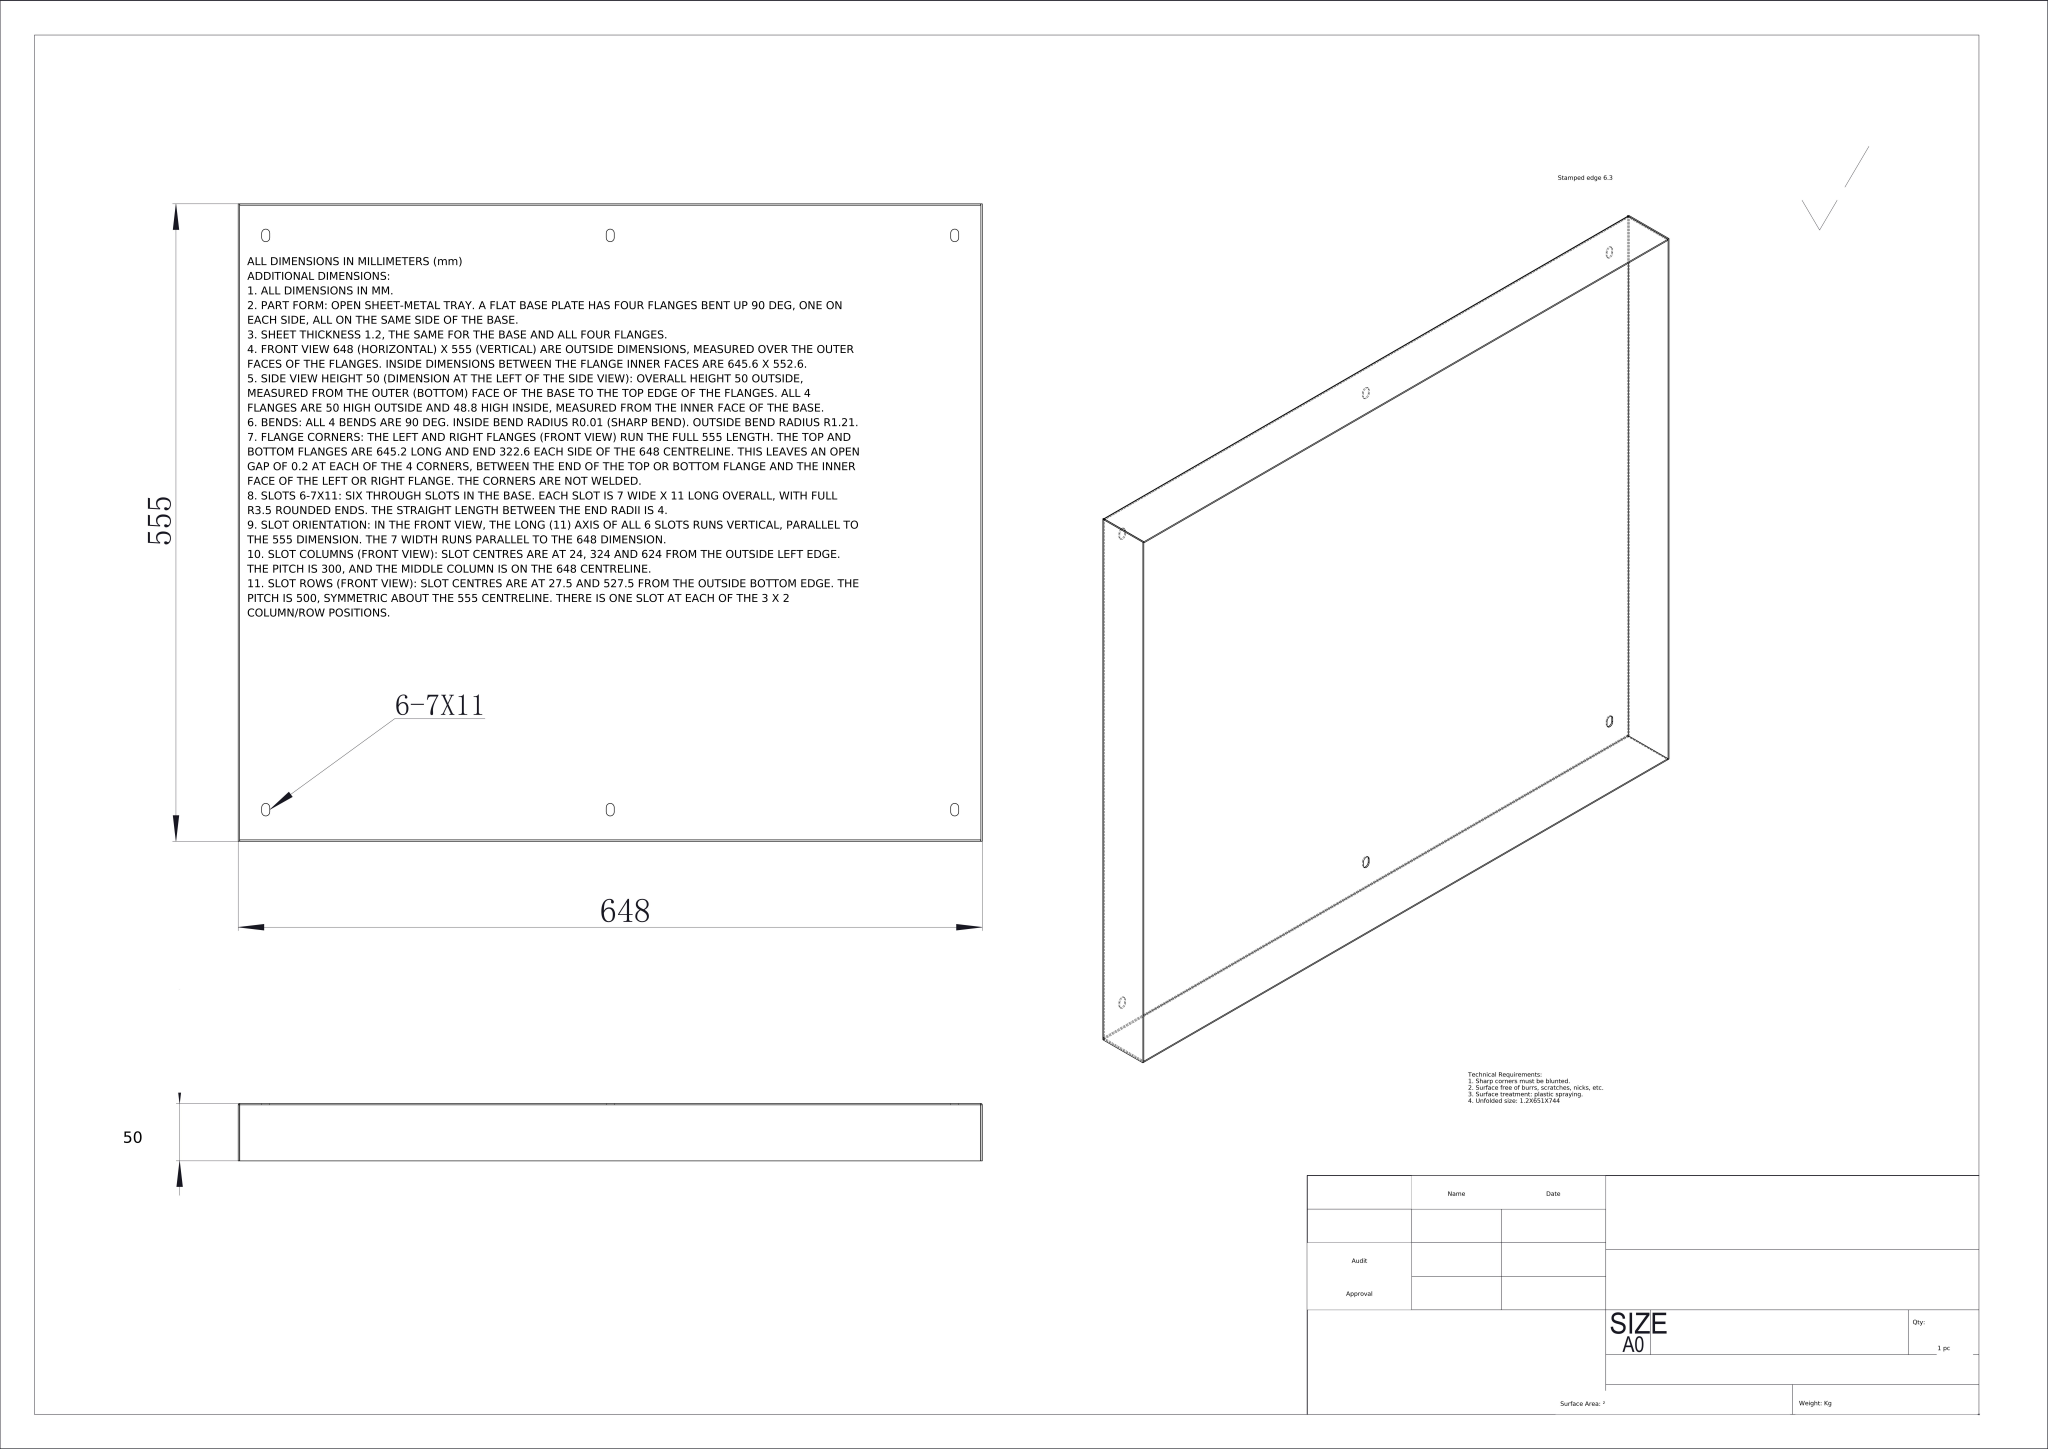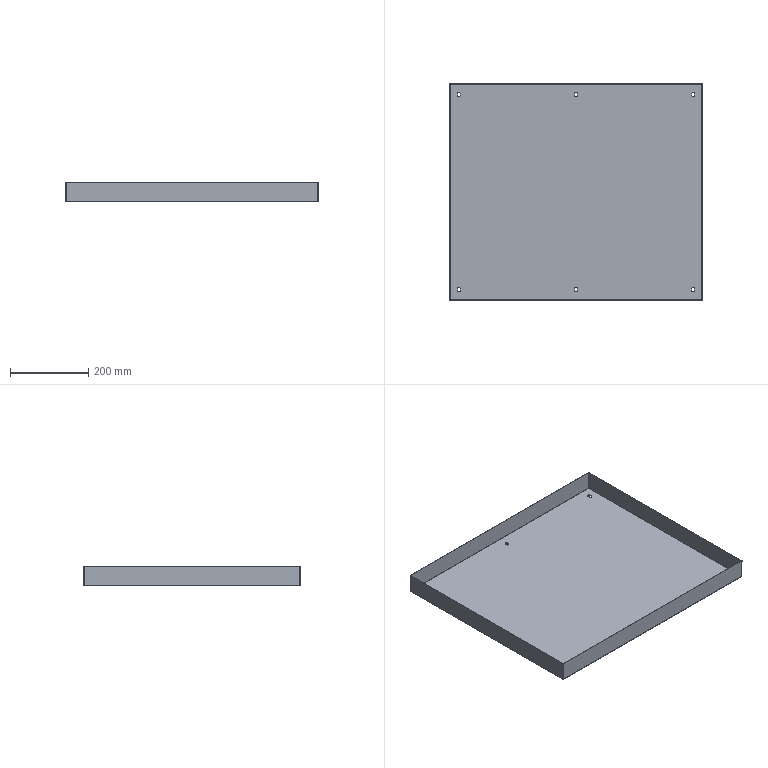Part | NX | mm | 1 solid | 78 faces | box 648 x 555 x 50 mm | volume 570902 mm3 | plane 58 | cylinder 20 | commonest cylinder face diameters 7 x12 2.42 x4 0.02 x4